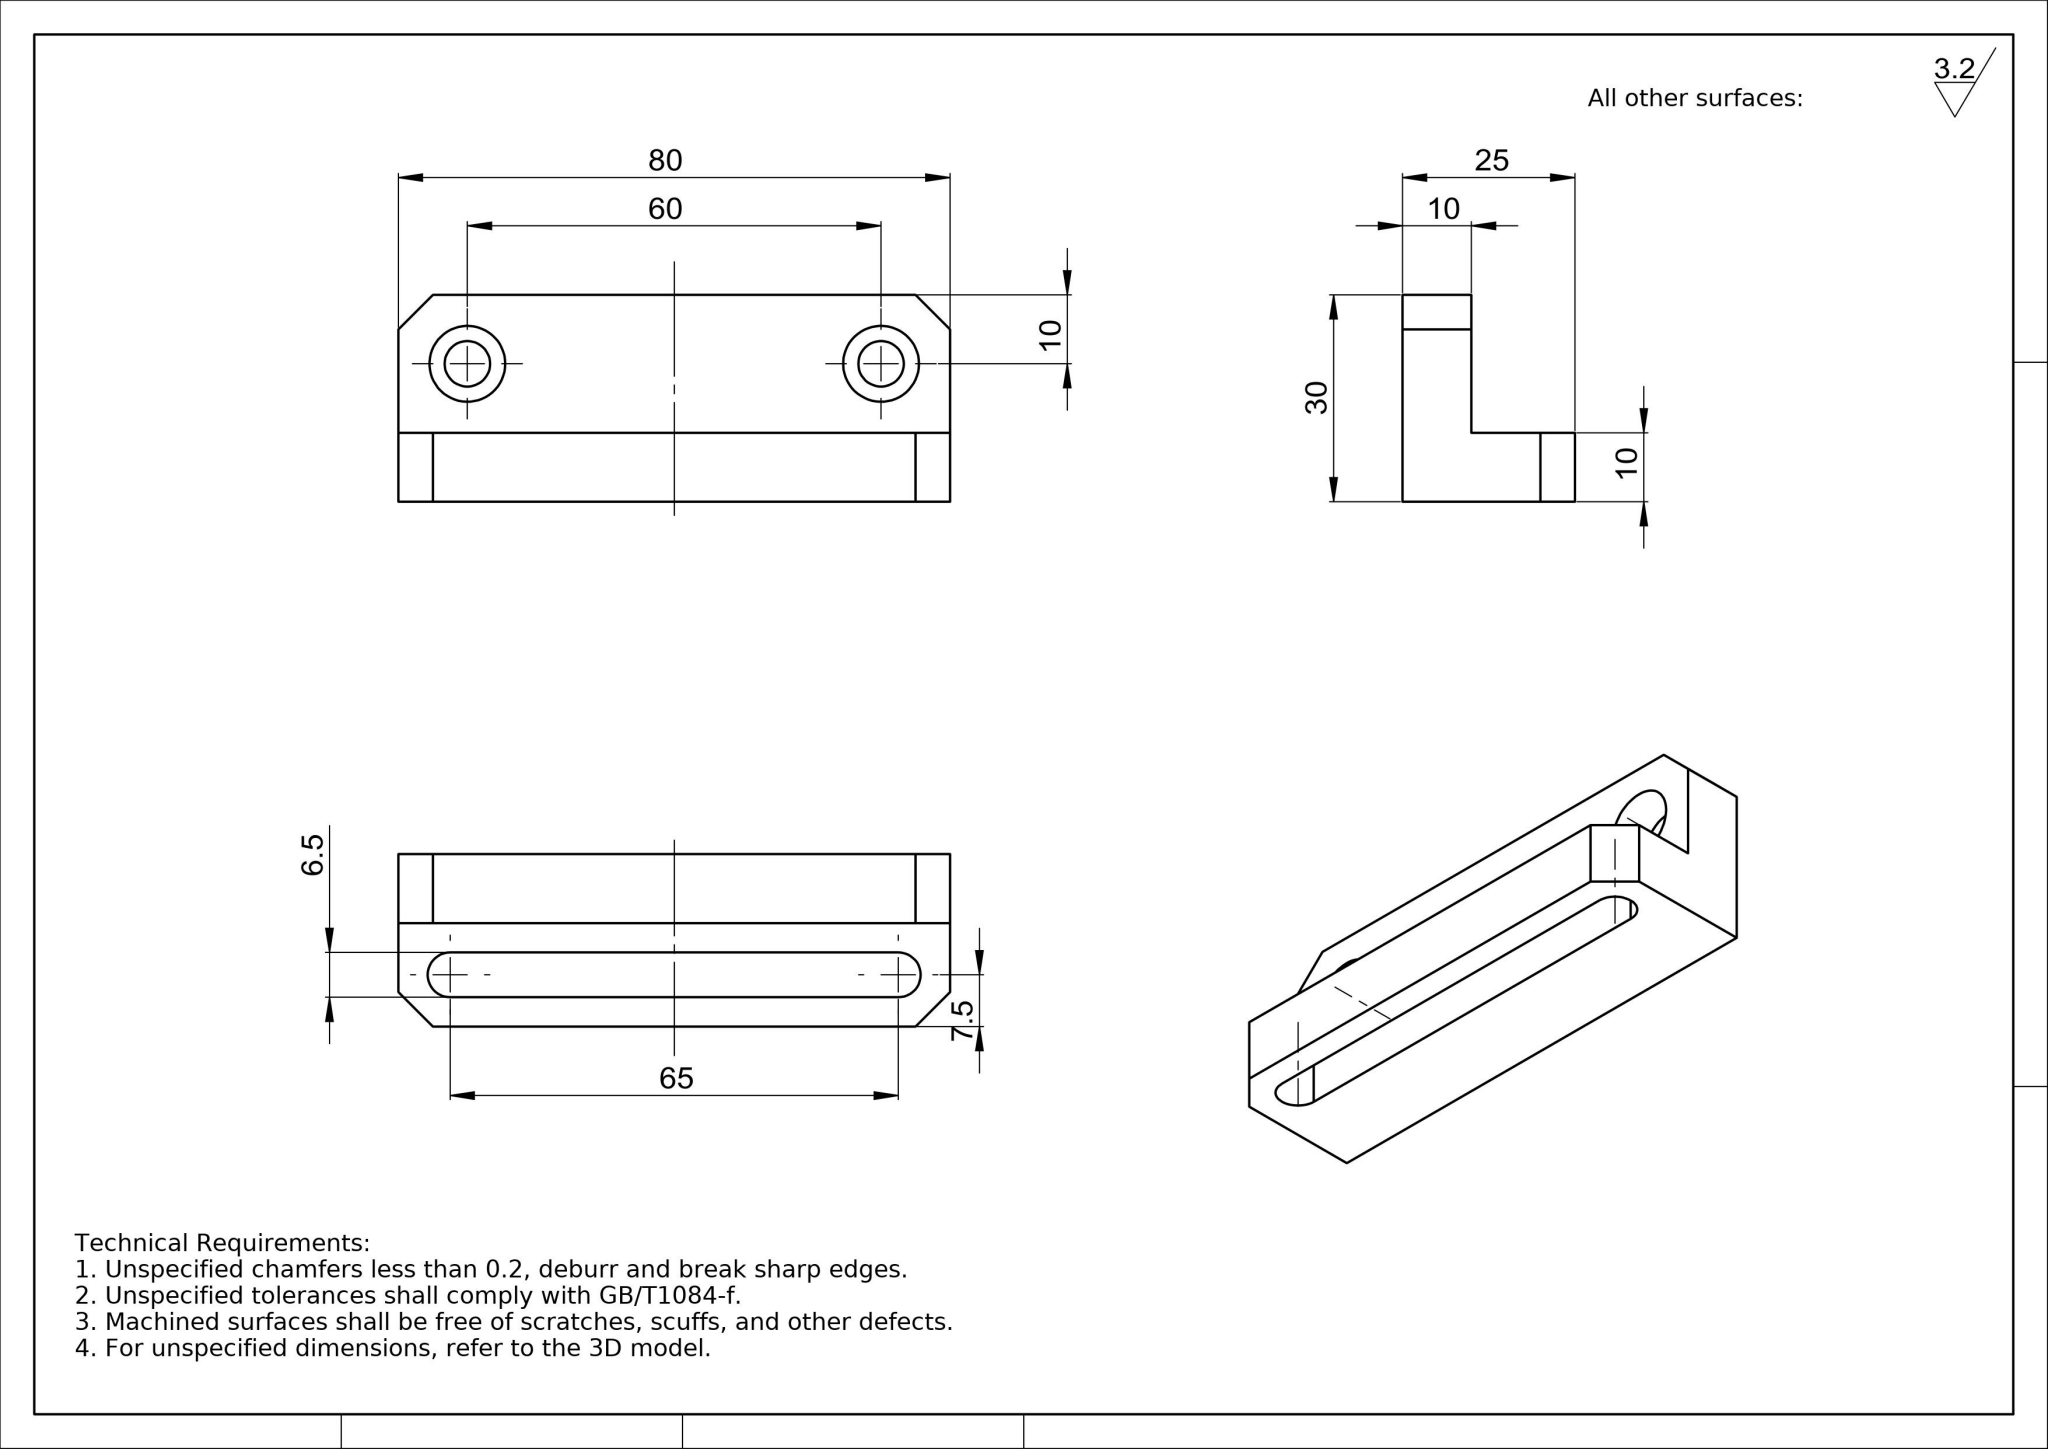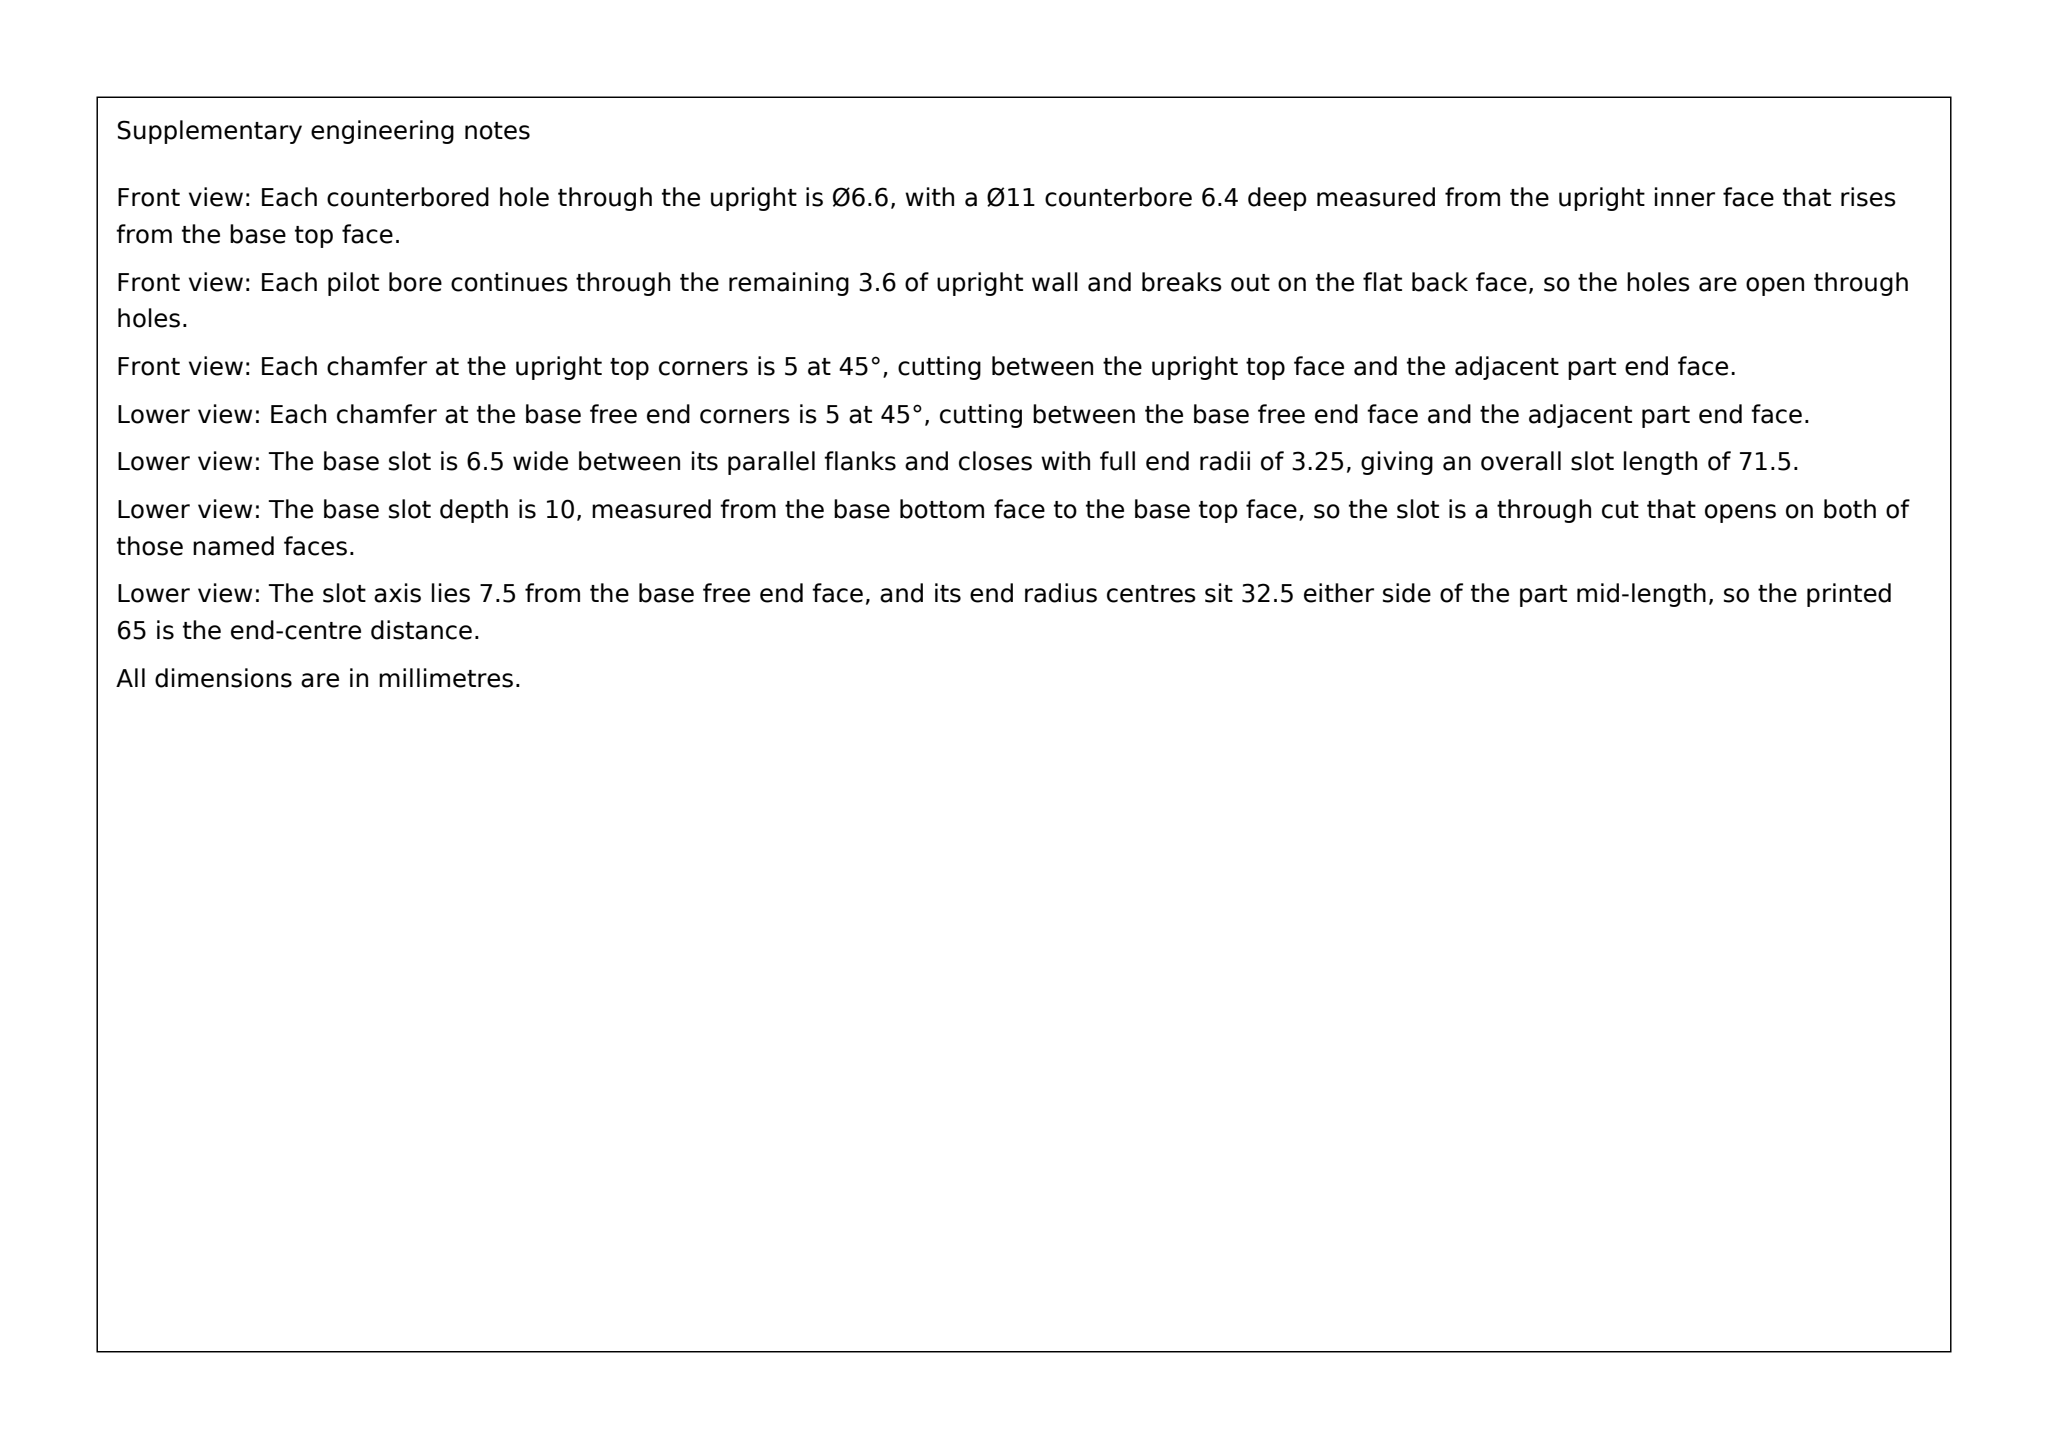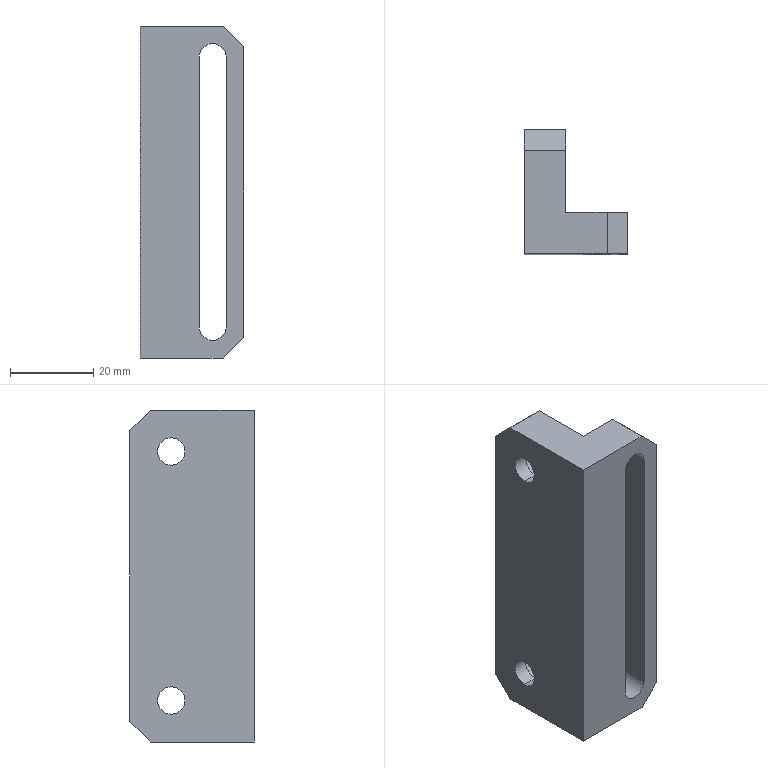Part | SolidWorks | mm | 1 solid | 26 faces | box 25 x 30 x 80 mm | volume 29480 mm3 | plane 16 | cylinder 10 | commonest cylinder face diameters 11 x4 6.6 x4 6.5 x2
Drawing notes:
SLOT 6.5 WIDE x 65 LG THRU 10 THK BASE | from the solid: Ø6.5 y-axis cyls at z=7.5 & 72.5 (65 apart), len 10 = y0 to y10 plate
2X Ø6.6 THRU, CBORE Ø11 DP 6.4 (CBORE, FLAT BTM) IN FRONT FACE | from the solid: Ø6.6 x 3.6 deep thru remaining wall + coaxial Ø11 x 6.4 flat-bottom bore, axis X, at y=20, z=10 & z=70 (10 wall)
build123d program:
from build123d import *

# Parameters (mm, degrees)
BOSS_EXTRUDE1_DEPTH                             = 40
CHAMFER1_SIZE                                   = 5
M6_HEX_SOCKET_HEAD_CAP_SCREW_CBORE1_D           = 6.6
M6_HEX_SOCKET_HEAD_CAP_SCREW_CBORE1_DEPTH       = 17.4
M6_HEX_SOCKET_HEAD_CAP_SCREW_CBORE1_CBORE_D     = 11
M6_HEX_SOCKET_HEAD_CAP_SCREW_CBORE1_CBORE_DEPTH = 6.4
M6_HEX_SOCKET_HEAD_CAP_SCREW_CBORE1_TIP         = 1.983
CUT_EXTRUDE1_DEPTH                              = 52.235


with BuildPart() as part:
    # Sketch1 → Boss-Extrude1 (new, symmetric)
    with BuildSketch(Plane.XY):
        Polygon((0, 0), (0, 30), (10, 30), (10, 10), (25, 10), (25, 0), align=None)
    extrude(amount=BOSS_EXTRUDE1_DEPTH, both=True)

    # Chamfer1
    chamfer1_edges = [part.edges().sort_by_distance(p)[0] for p in [
        (5, 30, 40),
        (5, 30, -40),
        (25, 5, -40),
        (25, 5, 40),
    ]]
    chamfer(chamfer1_edges, length=CHAMFER1_SIZE)

    # M6 Hex Socket Head Cap Screw CBORE1
    with Locations(Plane(origin=(10, 0, 0), x_dir=(0, 0, -1), z_dir=(1, 0, 0))):
        with Locations((-30, 20), (30, 20)):
            CounterBoreHole(M6_HEX_SOCKET_HEAD_CAP_SCREW_CBORE1_D / 2, M6_HEX_SOCKET_HEAD_CAP_SCREW_CBORE1_CBORE_D / 2, M6_HEX_SOCKET_HEAD_CAP_SCREW_CBORE1_CBORE_DEPTH, depth=M6_HEX_SOCKET_HEAD_CAP_SCREW_CBORE1_DEPTH)
            with Locations((0, 0, -(M6_HEX_SOCKET_HEAD_CAP_SCREW_CBORE1_DEPTH + M6_HEX_SOCKET_HEAD_CAP_SCREW_CBORE1_TIP / 2))):  # 118° drill point
                Cone(0, M6_HEX_SOCKET_HEAD_CAP_SCREW_CBORE1_D / 2, M6_HEX_SOCKET_HEAD_CAP_SCREW_CBORE1_TIP, mode=Mode.SUBTRACT)

    # Sketch4 → Cut-Extrude1 (cut, through all)
    with BuildSketch(Plane(origin=(0, 10, 0), x_dir=(1, 0, 0), z_dir=(0, 1, 0))):
        with BuildLine():
            Line((20.75, 32.5), (20.75, -32.5))
            ThreePointArc((20.75, -32.5), (17.5, -35.75), (14.25, -32.5))
            Line((14.25, -32.5), (14.25, 32.5))
            ThreePointArc((14.25, 32.5), (17.5, 35.75), (20.75, 32.5))
        make_face()
    extrude(amount=-CUT_EXTRUDE1_DEPTH, mode=Mode.SUBTRACT)


solid = part.part
STEP:
#1=CARTESIAN_POINT('',(3.6,20.,35.5));
#2=VERTEX_POINT('',#1);
#3=CARTESIAN_POINT('',(3.6,20.,24.5));
#4=VERTEX_POINT('',#3);
#5=CARTESIAN_POINT('',(3.6,20.,30.));
#6=DIRECTION('',(1.,0.,0.));
#7=DIRECTION('',(0.,0.,-1.));
#8=AXIS2_PLACEMENT_3D('',#5,#6,#7);
#9=CIRCLE('',#8,5.5);
#10=EDGE_CURVE('',#2,#4,#9,.T.);
#11=ORIENTED_EDGE('',*,*,#10,.F.);
#12=CARTESIAN_POINT('',(10.,20.,35.5));
#13=VERTEX_POINT('',#12);
#14=CARTESIAN_POINT('',(10.,20.,35.5));
#15=DIRECTION('',(1.,0.,0.));
#16=VECTOR('',#15,1000.);
#17=LINE('',#14,#16);
#18=EDGE_CURVE('',#2,#13,#17,.T.);
#19=ORIENTED_EDGE('',*,*,#18,.T.);
#20=CARTESIAN_POINT('',(10.,20.,24.5));
#21=VERTEX_POINT('',#20);
#22=CARTESIAN_POINT('',(10.,20.,30.));
#23=DIRECTION('',(1.,0.,0.));
#24=DIRECTION('',(0.,0.,-1.));
#25=AXIS2_PLACEMENT_3D('',#22,#23,#24);
#26=CIRCLE('',#25,5.5);
#27=EDGE_CURVE('',#13,#21,#26,.T.);
#28=ORIENTED_EDGE('',*,*,#27,.T.);
#29=CARTESIAN_POINT('',(10.,20.,24.5));
#30=DIRECTION('',(1.,0.,0.));
#31=VECTOR('',#30,1000.);
#32=LINE('',#29,#31);
#33=EDGE_CURVE('',#4,#21,#32,.T.);
#34=ORIENTED_EDGE('',*,*,#33,.F.);
#35=EDGE_LOOP('',(#11,#19,#28,#34));
#36=FACE_OUTER_BOUND('',#35,.T.);
#37=CARTESIAN_POINT('',(10.,20.,30.));
#38=DIRECTION('',(1.,0.,0.));
#39=DIRECTION('',(0.,0.,-1.));
#40=AXIS2_PLACEMENT_3D('',#37,#38,#39);
#41=CYLINDRICAL_SURFACE('',#40,5.5);
#42=ADVANCED_FACE('',(#36),#41,.F.);
#43=CARTESIAN_POINT('',(0.,20.,33.3));
#44=VERTEX_POINT('',#43);
#45=CARTESIAN_POINT('',(0.,20.,26.7));
#46=VERTEX_POINT('',#45);
#47=CARTESIAN_POINT('',(0.,20.,30.));
#48=DIRECTION('',(1.,0.,0.));
#49=DIRECTION('',(0.,0.,-1.));
#50=AXIS2_PLACEMENT_3D('',#47,#48,#49);
#51=CIRCLE('',#50,3.3);
#52=EDGE_CURVE('',#44,#46,#51,.T.);
#53=ORIENTED_EDGE('',*,*,#52,.F.);
#54=CARTESIAN_POINT('',(3.6,20.,33.3));
#55=VERTEX_POINT('',#54);
#56=CARTESIAN_POINT('',(10.,20.,33.3));
#57=DIRECTION('',(1.,0.,0.));
#58=VECTOR('',#57,1000.);
#59=LINE('',#56,#58);
#60=EDGE_CURVE('',#44,#55,#59,.T.);
#61=ORIENTED_EDGE('',*,*,#60,.T.);
#62=CARTESIAN_POINT('',(3.6,20.,26.7));
#63=VERTEX_POINT('',#62);
#64=CARTESIAN_POINT('',(3.6,20.,30.));
#65=DIRECTION('',(1.,0.,0.));
#66=DIRECTION('',(0.,0.,-1.));
#67=AXIS2_PLACEMENT_3D('',#64,#65,#66);
#68=CIRCLE('',#67,3.3);
#69=EDGE_CURVE('',#55,#63,#68,.T.);
#70=ORIENTED_EDGE('',*,*,#69,.T.);
#71=CARTESIAN_POINT('',(10.,20.,26.7));
#72=DIRECTION('',(1.,0.,0.));
#73=VECTOR('',#72,1000.);
#74=LINE('',#71,#73);
#75=EDGE_CURVE('',#46,#63,#74,.T.);
#76=ORIENTED_EDGE('',*,*,#75,.F.);
#77=EDGE_LOOP('',(#53,#61,#70,#76));
#78=FACE_OUTER_BOUND('',#77,.T.);
#79=CARTESIAN_POINT('',(10.,20.,30.));
#80=DIRECTION('',(1.,0.,0.));
#81=DIRECTION('',(0.,0.,-1.));
#82=AXIS2_PLACEMENT_3D('',#79,#80,#81);
#83=CYLINDRICAL_SURFACE('',#82,3.3);
#84=ADVANCED_FACE('',(#78),#83,.F.);
#85=CARTESIAN_POINT('',(3.6,20.,-24.5));
#86=VERTEX_POINT('',#85);
#87=CARTESIAN_POINT('',(3.6,20.,-35.5));
#88=VERTEX_POINT('',#87);
#89=CARTESIAN_POINT('',(3.6,20.,-30.));
#90=DIRECTION('',(1.,0.,0.));
#91=DIRECTION('',(0.,0.,-1.));
#92=AXIS2_PLACEMENT_3D('',#89,#90,#91);
#93=CIRCLE('',#92,5.5);
#94=EDGE_CURVE('',#86,#88,#93,.T.);
#95=ORIENTED_EDGE('',*,*,#94,.F.);
#96=CARTESIAN_POINT('',(10.,20.,-24.5));
#97=VERTEX_POINT('',#96);
#98=CARTESIAN_POINT('',(10.,20.,-24.5));
#99=DIRECTION('',(1.,0.,0.));
#100=VECTOR('',#99,1000.);
#101=LINE('',#98,#100);
#102=EDGE_CURVE('',#86,#97,#101,.T.);
#103=ORIENTED_EDGE('',*,*,#102,.T.);
#104=CARTESIAN_POINT('',(10.,20.,-35.5));
#105=VERTEX_POINT('',#104);
#106=CARTESIAN_POINT('',(10.,20.,-30.));
#107=DIRECTION('',(1.,0.,0.));
#108=DIRECTION('',(0.,0.,-1.));
#109=AXIS2_PLACEMENT_3D('',#106,#107,#108);
#110=CIRCLE('',#109,5.5);
#111=EDGE_CURVE('',#97,#105,#110,.T.);
#112=ORIENTED_EDGE('',*,*,#111,.T.);
#113=CARTESIAN_POINT('',(10.,20.,-35.5));
#114=DIRECTION('',(1.,0.,0.));
#115=VECTOR('',#114,1000.);
#116=LINE('',#113,#115);
#117=EDGE_CURVE('',#88,#105,#116,.T.);
#118=ORIENTED_EDGE('',*,*,#117,.F.);
#119=EDGE_LOOP('',(#95,#103,#112,#118));
#120=FACE_OUTER_BOUND('',#119,.T.);
#121=CARTESIAN_POINT('',(10.,20.,-30.));
#122=DIRECTION('',(1.,0.,0.));
#123=DIRECTION('',(0.,0.,-1.));
#124=AXIS2_PLACEMENT_3D('',#121,#122,#123);
#125=CYLINDRICAL_SURFACE('',#124,5.5);
#126=ADVANCED_FACE('',(#120),#125,.F.);
#127=CARTESIAN_POINT('',(0.,20.,-26.7));
#128=VERTEX_POINT('',#127);
#129=CARTESIAN_POINT('',(0.,20.,-33.3));
#130=VERTEX_POINT('',#129);
#131=CARTESIAN_POINT('',(0.,20.,-30.));
#132=DIRECTION('',(1.,0.,0.));
#133=DIRECTION('',(0.,0.,-1.));
#134=AXIS2_PLACEMENT_3D('',#131,#132,#133);
#135=CIRCLE('',#134,3.3);
#136=EDGE_CURVE('',#128,#130,#135,.T.);
#137=ORIENTED_EDGE('',*,*,#136,.F.);
#138=CARTESIAN_POINT('',(3.6,20.,-26.7));
#139=VERTEX_POINT('',#138);
#140=CARTESIAN_POINT('',(10.,20.,-26.7));
#141=DIRECTION('',(1.,0.,0.));
#142=VECTOR('',#141,1000.);
#143=LINE('',#140,#142);
#144=EDGE_CURVE('',#128,#139,#143,.T.);
#145=ORIENTED_EDGE('',*,*,#144,.T.);
#146=CARTESIAN_POINT('',(3.6,20.,-33.3));
#147=VERTEX_POINT('',#146);
#148=CARTESIAN_POINT('',(3.6,20.,-30.));
#149=DIRECTION('',(1.,0.,0.));
#150=DIRECTION('',(0.,0.,-1.));
#151=AXIS2_PLACEMENT_3D('',#148,#149,#150);
#152=CIRCLE('',#151,3.3);
#153=EDGE_CURVE('',#139,#147,#152,.T.);
#154=ORIENTED_EDGE('',*,*,#153,.T.);
#155=CARTESIAN_POINT('',(10.,20.,-33.3));
#156=DIRECTION('',(1.,0.,0.));
#157=VECTOR('',#156,1000.);
#158=LINE('',#155,#157);
#159=EDGE_CURVE('',#130,#147,#158,.T.);
#160=ORIENTED_EDGE('',*,*,#159,.F.);
#161=EDGE_LOOP('',(#137,#145,#154,#160));
#162=FACE_OUTER_BOUND('',#161,.T.);
#163=CARTESIAN_POINT('',(10.,20.,-30.));
#164=DIRECTION('',(1.,0.,0.));
#165=DIRECTION('',(0.,0.,-1.));
#166=AXIS2_PLACEMENT_3D('',#163,#164,#165);
#167=CYLINDRICAL_SURFACE('',#166,3.3);
#168=ADVANCED_FACE('',(#162),#167,.F.);
#169=CARTESIAN_POINT('',(20.75,-0.,32.5));
#170=VERTEX_POINT('',#169);
#171=CARTESIAN_POINT('',(20.75,-0.,-32.5));
#172=VERTEX_POINT('',#171);
#173=CARTESIAN_POINT('',(20.75,-0.,-32.5));
#174=DIRECTION('',(0.,0.,-1.));
#175=VECTOR('',#174,1000.);
#176=LINE('',#173,#175);
#177=EDGE_CURVE('',#170,#172,#176,.T.);
#178=ORIENTED_EDGE('',*,*,#177,.T.);
#179=CARTESIAN_POINT('',(14.25,-0.,-32.5));
#180=VERTEX_POINT('',#179);
#181=CARTESIAN_POINT('',(17.5,-0.,-32.5));
#182=DIRECTION('',(0.,1.,0.));
#183=DIRECTION('',(-1.,0.,0.));
#184=AXIS2_PLACEMENT_3D('',#181,#182,#183);
#185=CIRCLE('',#184,3.25);
#186=EDGE_CURVE('',#172,#180,#185,.T.);
#187=ORIENTED_EDGE('',*,*,#186,.T.);
#188=CARTESIAN_POINT('',(14.25,0.,32.5));
#189=VERTEX_POINT('',#188);
#190=CARTESIAN_POINT('',(14.25,-0.,-32.5));
#191=DIRECTION('',(0.,0.,1.));
#192=VECTOR('',#191,1000.);
#193=LINE('',#190,#192);
#194=EDGE_CURVE('',#180,#189,#193,.T.);
#195=ORIENTED_EDGE('',*,*,#194,.T.);
#196=CARTESIAN_POINT('',(17.5,-0.,32.5));
#197=DIRECTION('',(0.,1.,0.));
#198=DIRECTION('',(-1.,0.,0.));
#199=AXIS2_PLACEMENT_3D('',#196,#197,#198);
#200=CIRCLE('',#199,3.25);
#201=EDGE_CURVE('',#189,#170,#200,.T.);
#202=ORIENTED_EDGE('',*,*,#201,.T.);
#203=EDGE_LOOP('',(#178,#187,#195,#202));
#204=FACE_BOUND('',#203,.T.);
#205=CARTESIAN_POINT('',(0.,0.,-40.));
#206=VERTEX_POINT('',#205);
#207=CARTESIAN_POINT('',(20.,0.,-40.));
#208=VERTEX_POINT('',#207);
#209=CARTESIAN_POINT('',(25.,0.,-40.));
#210=DIRECTION('',(1.,0.,0.));
#211=VECTOR('',#210,1000.);
#212=LINE('',#209,#211);
#213=EDGE_CURVE('',#206,#208,#212,.T.);
#214=ORIENTED_EDGE('',*,*,#213,.T.);
#215=CARTESIAN_POINT('',(25.,0.,-35.));
#216=VERTEX_POINT('',#215);
#217=CARTESIAN_POINT('',(25.,0.,-35.));
#218=DIRECTION('',(0.7071,0.,0.7071));
#219=VECTOR('',#218,1000.);
#220=LINE('',#217,#219);
#221=EDGE_CURVE('',#208,#216,#220,.T.);
#222=ORIENTED_EDGE('',*,*,#221,.T.);
#223=CARTESIAN_POINT('',(25.,0.,35.));
#224=VERTEX_POINT('',#223);
#225=CARTESIAN_POINT('',(25.,0.,40.));
#226=DIRECTION('',(0.,0.,-1.));
#227=VECTOR('',#226,1000.);
#228=LINE('',#225,#227);
#229=EDGE_CURVE('',#224,#216,#228,.T.);
#230=ORIENTED_EDGE('',*,*,#229,.F.);
#231=CARTESIAN_POINT('',(20.,0.,40.));
#232=VERTEX_POINT('',#231);
#233=CARTESIAN_POINT('',(20.,0.,40.));
#234=DIRECTION('',(-0.7071,-0.,0.7071));
#235=VECTOR('',#234,1000.);
#236=LINE('',#233,#235);
#237=EDGE_CURVE('',#224,#232,#236,.T.);
#238=ORIENTED_EDGE('',*,*,#237,.T.);
#239=CARTESIAN_POINT('',(0.,0.,40.));
#240=VERTEX_POINT('',#239);
#241=CARTESIAN_POINT('',(25.,0.,40.));
#242=DIRECTION('',(1.,0.,0.));
#243=VECTOR('',#242,1000.);
#244=LINE('',#241,#243);
#245=EDGE_CURVE('',#240,#232,#244,.T.);
#246=ORIENTED_EDGE('',*,*,#245,.F.);
#247=CARTESIAN_POINT('',(0.,0.,40.));
#248=DIRECTION('',(0.,0.,-1.));
#249=VECTOR('',#248,1000.);
#250=LINE('',#247,#249);
#251=EDGE_CURVE('',#240,#206,#250,.T.);
#252=ORIENTED_EDGE('',*,*,#251,.T.);
#253=EDGE_LOOP('',(#214,#222,#230,#238,#246,#252));
#254=FACE_OUTER_BOUND('',#253,.T.);
#255=CARTESIAN_POINT('',(25.,0.,40.));
#256=DIRECTION('',(-0.,1.,0.));
#257=DIRECTION('',(-1.,-0.,0.));
#258=AXIS2_PLACEMENT_3D('',#255,#256,#257);
#259=PLANE('',#258);
#260=ADVANCED_FACE('',(#204,#254),#259,.F.);
#261=ORIENTED_EDGE('',*,*,#229,.T.);
#262=CARTESIAN_POINT('',(25.,10.,-35.));
#263=VERTEX_POINT('',#262);
#264=CARTESIAN_POINT('',(25.,10.,-35.));
#265=DIRECTION('',(0.,1.,0.));
#266=VECTOR('',#265,1000.);
#267=LINE('',#264,#266);
#268=EDGE_CURVE('',#216,#263,#267,.T.);
#269=ORIENTED_EDGE('',*,*,#268,.T.);
#270=CARTESIAN_POINT('',(25.,10.,35.));
#271=VERTEX_POINT('',#270);
#272=CARTESIAN_POINT('',(25.,10.,40.));
#273=DIRECTION('',(0.,0.,-1.));
#274=VECTOR('',#273,1000.);
#275=LINE('',#272,#274);
#276=EDGE_CURVE('',#271,#263,#275,.T.);
#277=ORIENTED_EDGE('',*,*,#276,.F.);
#278=CARTESIAN_POINT('',(25.,10.,35.));
#279=DIRECTION('',(0.,-1.,0.));
#280=VECTOR('',#279,1000.);
#281=LINE('',#278,#280);
#282=EDGE_CURVE('',#271,#224,#281,.T.);
#283=ORIENTED_EDGE('',*,*,#282,.T.);
#284=EDGE_LOOP('',(#261,#269,#277,#283));
#285=FACE_OUTER_BOUND('',#284,.T.);
#286=CARTESIAN_POINT('',(25.,10.,40.));
#287=DIRECTION('',(-1.,0.,0.));
#288=DIRECTION('',(0.,0.,1.));
#289=AXIS2_PLACEMENT_3D('',#286,#287,#288);
#290=PLANE('',#289);
#291=ADVANCED_FACE('',(#285),#290,.F.);
#292=CARTESIAN_POINT('',(14.25,10.,-32.5));
#293=VERTEX_POINT('',#292);
#294=CARTESIAN_POINT('',(14.25,10.,32.5));
#295=VERTEX_POINT('',#294);
#296=CARTESIAN_POINT('',(14.25,10.,-32.5));
#297=DIRECTION('',(0.,0.,1.));
#298=VECTOR('',#297,1000.);
#299=LINE('',#296,#298);
#300=EDGE_CURVE('',#293,#295,#299,.T.);
#301=ORIENTED_EDGE('',*,*,#300,.F.);
#302=CARTESIAN_POINT('',(20.75,10.,-32.5));
#303=VERTEX_POINT('',#302);
#304=CARTESIAN_POINT('',(17.5,10.,-32.5));
#305=DIRECTION('',(0.,1.,0.));
#306=DIRECTION('',(-1.,0.,0.));
#307=AXIS2_PLACEMENT_3D('',#304,#305,#306);
#308=CIRCLE('',#307,3.25);
#309=EDGE_CURVE('',#303,#293,#308,.T.);
#310=ORIENTED_EDGE('',*,*,#309,.F.);
#311=CARTESIAN_POINT('',(20.75,10.,32.5));
#312=VERTEX_POINT('',#311);
#313=CARTESIAN_POINT('',(20.75,10.,-32.5));
#314=DIRECTION('',(0.,0.,-1.));
#315=VECTOR('',#314,1000.);
#316=LINE('',#313,#315);
#317=EDGE_CURVE('',#312,#303,#316,.T.);
#318=ORIENTED_EDGE('',*,*,#317,.F.);
#319=CARTESIAN_POINT('',(17.5,10.,32.5));
#320=DIRECTION('',(0.,1.,0.));
#321=DIRECTION('',(-1.,0.,0.));
#322=AXIS2_PLACEMENT_3D('',#319,#320,#321);
#323=CIRCLE('',#322,3.25);
#324=EDGE_CURVE('',#295,#312,#323,.T.);
#325=ORIENTED_EDGE('',*,*,#324,.F.);
#326=EDGE_LOOP('',(#301,#310,#318,#325));
#327=FACE_BOUND('',#326,.T.);
#328=ORIENTED_EDGE('',*,*,#276,.T.);
#329=CARTESIAN_POINT('',(20.,10.,-40.));
#330=VERTEX_POINT('',#329);
#331=CARTESIAN_POINT('',(25.,10.,-35.));
#332=DIRECTION('',(-0.7071,0.,-0.7071));
#333=VECTOR('',#332,1000.);
#334=LINE('',#331,#333);
#335=EDGE_CURVE('',#263,#330,#334,.T.);
#336=ORIENTED_EDGE('',*,*,#335,.T.);
#337=CARTESIAN_POINT('',(10.,10.,-40.));
#338=VERTEX_POINT('',#337);
#339=CARTESIAN_POINT('',(10.,10.,-40.));
#340=DIRECTION('',(-1.,0.,0.));
#341=VECTOR('',#340,1000.);
#342=LINE('',#339,#341);
#343=EDGE_CURVE('',#330,#338,#342,.T.);
#344=ORIENTED_EDGE('',*,*,#343,.T.);
#345=CARTESIAN_POINT('',(10.,10.,40.));
#346=VERTEX_POINT('',#345);
#347=CARTESIAN_POINT('',(10.,10.,40.));
#348=DIRECTION('',(0.,0.,-1.));
#349=VECTOR('',#348,1000.);
#350=LINE('',#347,#349);
#351=EDGE_CURVE('',#346,#338,#350,.T.);
#352=ORIENTED_EDGE('',*,*,#351,.F.);
#353=CARTESIAN_POINT('',(20.,10.,40.));
#354=VERTEX_POINT('',#353);
#355=CARTESIAN_POINT('',(10.,10.,40.));
#356=DIRECTION('',(-1.,0.,0.));
#357=VECTOR('',#356,1000.);
#358=LINE('',#355,#357);
#359=EDGE_CURVE('',#354,#346,#358,.T.);
#360=ORIENTED_EDGE('',*,*,#359,.F.);
#361=CARTESIAN_POINT('',(20.,10.,40.));
#362=DIRECTION('',(0.7071,-0.,-0.7071));
#363=VECTOR('',#362,1000.);
#364=LINE('',#361,#363);
#365=EDGE_CURVE('',#354,#271,#364,.T.);
#366=ORIENTED_EDGE('',*,*,#365,.T.);
#367=EDGE_LOOP('',(#328,#336,#344,#352,#360,#366));
#368=FACE_OUTER_BOUND('',#367,.T.);
#369=CARTESIAN_POINT('',(10.,10.,40.));
#370=DIRECTION('',(-0.,-1.,0.));
#371=DIRECTION('',(1.,-0.,0.));
#372=AXIS2_PLACEMENT_3D('',#369,#370,#371);
#373=PLANE('',#372);
#374=ADVANCED_FACE('',(#327,#368),#373,.F.);
#375=CARTESIAN_POINT('',(10.,20.,30.));
#376=DIRECTION('',(1.,0.,0.));
#377=DIRECTION('',(0.,0.,-1.));
#378=AXIS2_PLACEMENT_3D('',#375,#376,#377);
#379=CIRCLE('',#378,5.5);
#380=EDGE_CURVE('',#21,#13,#379,.T.);
#381=ORIENTED_EDGE('',*,*,#380,.F.);
#382=ORIENTED_EDGE('',*,*,#27,.F.);
#383=EDGE_LOOP('',(#381,#382));
#384=FACE_BOUND('',#383,.T.);
#385=CARTESIAN_POINT('',(10.,20.,-30.));
#386=DIRECTION('',(1.,0.,0.));
#387=DIRECTION('',(0.,0.,-1.));
#388=AXIS2_PLACEMENT_3D('',#385,#386,#387);
#389=CIRCLE('',#388,5.5);
#390=EDGE_CURVE('',#105,#97,#389,.T.);
#391=ORIENTED_EDGE('',*,*,#390,.F.);
#392=ORIENTED_EDGE('',*,*,#111,.F.);
#393=EDGE_LOOP('',(#391,#392));
#394=FACE_BOUND('',#393,.T.);
#395=CARTESIAN_POINT('',(10.,25.,-40.));
#396=VERTEX_POINT('',#395);
#397=CARTESIAN_POINT('',(10.,30.,-40.));
#398=DIRECTION('',(0.,1.,0.));
#399=VECTOR('',#398,1000.);
#400=LINE('',#397,#399);
#401=EDGE_CURVE('',#338,#396,#400,.T.);
#402=ORIENTED_EDGE('',*,*,#401,.T.);
#403=CARTESIAN_POINT('',(10.,30.,-35.));
#404=VERTEX_POINT('',#403);
#405=CARTESIAN_POINT('',(10.,30.,-35.));
#406=DIRECTION('',(0.,0.7071,0.7071));
#407=VECTOR('',#406,1000.);
#408=LINE('',#405,#407);
#409=EDGE_CURVE('',#396,#404,#408,.T.);
#410=ORIENTED_EDGE('',*,*,#409,.T.);
#411=CARTESIAN_POINT('',(10.,30.,35.));
#412=VERTEX_POINT('',#411);
#413=CARTESIAN_POINT('',(10.,30.,40.));
#414=DIRECTION('',(0.,0.,-1.));
#415=VECTOR('',#414,1000.);
#416=LINE('',#413,#415);
#417=EDGE_CURVE('',#412,#404,#416,.T.);
#418=ORIENTED_EDGE('',*,*,#417,.F.);
#419=CARTESIAN_POINT('',(10.,25.,40.));
#420=VERTEX_POINT('',#419);
#421=CARTESIAN_POINT('',(10.,25.,40.));
#422=DIRECTION('',(0.,-0.7071,0.7071));
#423=VECTOR('',#422,1000.);
#424=LINE('',#421,#423);
#425=EDGE_CURVE('',#412,#420,#424,.T.);
#426=ORIENTED_EDGE('',*,*,#425,.T.);
#427=CARTESIAN_POINT('',(10.,30.,40.));
#428=DIRECTION('',(0.,1.,0.));
#429=VECTOR('',#428,1000.);
#430=LINE('',#427,#429);
#431=EDGE_CURVE('',#346,#420,#430,.T.);
#432=ORIENTED_EDGE('',*,*,#431,.F.);
#433=ORIENTED_EDGE('',*,*,#351,.T.);
#434=EDGE_LOOP('',(#402,#410,#418,#426,#432,#433));
#435=FACE_OUTER_BOUND('',#434,.T.);
#436=CARTESIAN_POINT('',(10.,30.,40.));
#437=DIRECTION('',(-1.,0.,0.));
#438=DIRECTION('',(0.,0.,1.));
#439=AXIS2_PLACEMENT_3D('',#436,#437,#438);
#440=PLANE('',#439);
#441=ADVANCED_FACE('',(#384,#394,#435),#440,.F.);
#442=ORIENTED_EDGE('',*,*,#417,.T.);
#443=CARTESIAN_POINT('',(0.,30.,-35.));
#444=VERTEX_POINT('',#443);
#445=CARTESIAN_POINT('',(0.,30.,-35.));
#446=DIRECTION('',(-1.,0.,0.));
#447=VECTOR('',#446,1000.);
#448=LINE('',#445,#447);
#449=EDGE_CURVE('',#404,#444,#448,.T.);
#450=ORIENTED_EDGE('',*,*,#449,.T.);
#451=CARTESIAN_POINT('',(0.,30.,35.));
#452=VERTEX_POINT('',#451);
#453=CARTESIAN_POINT('',(0.,30.,40.));
#454=DIRECTION('',(0.,0.,-1.));
#455=VECTOR('',#454,1000.);
#456=LINE('',#453,#455);
#457=EDGE_CURVE('',#452,#444,#456,.T.);
#458=ORIENTED_EDGE('',*,*,#457,.F.);
#459=CARTESIAN_POINT('',(0.,30.,35.));
#460=DIRECTION('',(1.,0.,0.));
#461=VECTOR('',#460,1000.);
#462=LINE('',#459,#461);
#463=EDGE_CURVE('',#452,#412,#462,.T.);
#464=ORIENTED_EDGE('',*,*,#463,.T.);
#465=EDGE_LOOP('',(#442,#450,#458,#464));
#466=FACE_OUTER_BOUND('',#465,.T.);
#467=CARTESIAN_POINT('',(0.,30.,40.));
#468=DIRECTION('',(0.,-1.,0.));
#469=DIRECTION('',(0.,0.,-1.));
#470=AXIS2_PLACEMENT_3D('',#467,#468,#469);
#471=PLANE('',#470);
#472=ADVANCED_FACE('',(#466),#471,.F.);
#473=CARTESIAN_POINT('',(0.,20.,30.));
#474=DIRECTION('',(1.,0.,0.));
#475=DIRECTION('',(0.,0.,-1.));
#476=AXIS2_PLACEMENT_3D('',#473,#474,#475);
#477=CIRCLE('',#476,3.3);
#478=EDGE_CURVE('',#46,#44,#477,.T.);
#479=ORIENTED_EDGE('',*,*,#478,.T.);
#480=ORIENTED_EDGE('',*,*,#52,.T.);
#481=EDGE_LOOP('',(#479,#480));
#482=FACE_BOUND('',#481,.T.);
#483=CARTESIAN_POINT('',(0.,20.,-30.));
#484=DIRECTION('',(1.,0.,0.));
#485=DIRECTION('',(0.,0.,-1.));
#486=AXIS2_PLACEMENT_3D('',#483,#484,#485);
#487=CIRCLE('',#486,3.3);
#488=EDGE_CURVE('',#130,#128,#487,.T.);
#489=ORIENTED_EDGE('',*,*,#488,.T.);
#490=ORIENTED_EDGE('',*,*,#136,.T.);
#491=EDGE_LOOP('',(#489,#490));
#492=FACE_BOUND('',#491,.T.);
#493=ORIENTED_EDGE('',*,*,#457,.T.);
#494=CARTESIAN_POINT('',(0.,25.,-40.));
#495=VERTEX_POINT('',#494);
#496=CARTESIAN_POINT('',(0.,30.,-35.));
#497=DIRECTION('',(0.,-0.7071,-0.7071));
#498=VECTOR('',#497,1000.);
#499=LINE('',#496,#498);
#500=EDGE_CURVE('',#444,#495,#499,.T.);
#501=ORIENTED_EDGE('',*,*,#500,.T.);
#502=CARTESIAN_POINT('',(0.,0.,-40.));
#503=DIRECTION('',(0.,-1.,0.));
#504=VECTOR('',#503,1000.);
#505=LINE('',#502,#504);
#506=EDGE_CURVE('',#495,#206,#505,.T.);
#507=ORIENTED_EDGE('',*,*,#506,.T.);
#508=ORIENTED_EDGE('',*,*,#251,.F.);
#509=CARTESIAN_POINT('',(0.,25.,40.));
#510=VERTEX_POINT('',#509);
#511=CARTESIAN_POINT('',(0.,0.,40.));
#512=DIRECTION('',(0.,-1.,0.));
#513=VECTOR('',#512,1000.);
#514=LINE('',#511,#513);
#515=EDGE_CURVE('',#510,#240,#514,.T.);
#516=ORIENTED_EDGE('',*,*,#515,.F.);
#517=CARTESIAN_POINT('',(0.,25.,40.));
#518=DIRECTION('',(0.,0.7071,-0.7071));
#519=VECTOR('',#518,1000.);
#520=LINE('',#517,#519);
#521=EDGE_CURVE('',#510,#452,#520,.T.);
#522=ORIENTED_EDGE('',*,*,#521,.T.);
#523=EDGE_LOOP('',(#493,#501,#507,#508,#516,#522));
#524=FACE_OUTER_BOUND('',#523,.T.);
#525=CARTESIAN_POINT('',(0.,0.,40.));
#526=DIRECTION('',(1.,0.,0.));
#527=DIRECTION('',(0.,0.,-1.));
#528=AXIS2_PLACEMENT_3D('',#525,#526,#527);
#529=PLANE('',#528);
#530=ADVANCED_FACE('',(#482,#492,#524),#529,.F.);
#531=ORIENTED_EDGE('',*,*,#245,.T.);
#532=CARTESIAN_POINT('',(20.,0.,40.));
#533=DIRECTION('',(0.,1.,0.));
#534=VECTOR('',#533,1000.);
#535=LINE('',#532,#534);
#536=EDGE_CURVE('',#232,#354,#535,.T.);
#537=ORIENTED_EDGE('',*,*,#536,.T.);
#538=ORIENTED_EDGE('',*,*,#359,.T.);
#539=ORIENTED_EDGE('',*,*,#431,.T.);
#540=CARTESIAN_POINT('',(0.,25.,40.));
#541=DIRECTION('',(-1.,0.,0.));
#542=VECTOR('',#541,1000.);
#543=LINE('',#540,#542);
#544=EDGE_CURVE('',#420,#510,#543,.T.);
#545=ORIENTED_EDGE('',*,*,#544,.T.);
#546=ORIENTED_EDGE('',*,*,#515,.T.);
#547=EDGE_LOOP('',(#531,#537,#538,#539,#545,#546));
#548=FACE_OUTER_BOUND('',#547,.T.);
#549=CARTESIAN_POINT('',(0.,0.,40.));
#550=DIRECTION('',(0.,0.,-1.));
#551=DIRECTION('',(-1.,0.,0.));
#552=AXIS2_PLACEMENT_3D('',#549,#550,#551);
#553=PLANE('',#552);
#554=ADVANCED_FACE('',(#548),#553,.F.);
#555=ORIENTED_EDGE('',*,*,#343,.F.);
#556=CARTESIAN_POINT('',(20.,0.,-40.));
#557=DIRECTION('',(0.,-1.,0.));
#558=VECTOR('',#557,1000.);
#559=LINE('',#556,#558);
#560=EDGE_CURVE('',#330,#208,#559,.T.);
#561=ORIENTED_EDGE('',*,*,#560,.T.);
#562=ORIENTED_EDGE('',*,*,#213,.F.);
#563=ORIENTED_EDGE('',*,*,#506,.F.);
#564=CARTESIAN_POINT('',(10.,25.,-40.));
#565=DIRECTION('',(1.,0.,0.));
#566=VECTOR('',#565,1000.);
#567=LINE('',#564,#566);
#568=EDGE_CURVE('',#495,#396,#567,.T.);
#569=ORIENTED_EDGE('',*,*,#568,.T.);
#570=ORIENTED_EDGE('',*,*,#401,.F.);
#571=EDGE_LOOP('',(#555,#561,#562,#563,#569,#570));
#572=FACE_OUTER_BOUND('',#571,.T.);
#573=CARTESIAN_POINT('',(0.,0.,-40.));
#574=DIRECTION('',(0.,0.,-1.));
#575=DIRECTION('',(-1.,0.,0.));
#576=AXIS2_PLACEMENT_3D('',#573,#574,#575);
#577=PLANE('',#576);
#578=ADVANCED_FACE('',(#572),#577,.T.);
#579=ORIENTED_EDGE('',*,*,#221,.F.);
#580=ORIENTED_EDGE('',*,*,#560,.F.);
#581=ORIENTED_EDGE('',*,*,#335,.F.);
#582=ORIENTED_EDGE('',*,*,#268,.F.);
#583=EDGE_LOOP('',(#579,#580,#581,#582));
#584=FACE_OUTER_BOUND('',#583,.T.);
#585=CARTESIAN_POINT('',(25.,10.,-35.));
#586=DIRECTION('',(0.7071,0.,-0.7071));
#587=DIRECTION('',(0.,-1.,0.));
#588=AXIS2_PLACEMENT_3D('',#585,#586,#587);
#589=PLANE('',#588);
#590=ADVANCED_FACE('',(#584),#589,.T.);
#591=ORIENTED_EDGE('',*,*,#237,.F.);
#592=ORIENTED_EDGE('',*,*,#282,.F.);
#593=ORIENTED_EDGE('',*,*,#365,.F.);
#594=ORIENTED_EDGE('',*,*,#536,.F.);
#595=EDGE_LOOP('',(#591,#592,#593,#594));
#596=FACE_OUTER_BOUND('',#595,.T.);
#597=CARTESIAN_POINT('',(20.,0.,40.));
#598=DIRECTION('',(-0.7071,0.,-0.7071));
#599=DIRECTION('',(0.,1.,0.));
#600=AXIS2_PLACEMENT_3D('',#597,#598,#599);
#601=PLANE('',#600);
#602=ADVANCED_FACE('',(#596),#601,.F.);
#603=ORIENTED_EDGE('',*,*,#409,.F.);
#604=ORIENTED_EDGE('',*,*,#568,.F.);
#605=ORIENTED_EDGE('',*,*,#500,.F.);
#606=ORIENTED_EDGE('',*,*,#449,.F.);
#607=EDGE_LOOP('',(#603,#604,#605,#606));
#608=FACE_OUTER_BOUND('',#607,.T.);
#609=CARTESIAN_POINT('',(0.,30.,-35.));
#610=DIRECTION('',(0.,0.7071,-0.7071));
#611=DIRECTION('',(1.,0.,0.));
#612=AXIS2_PLACEMENT_3D('',#609,#610,#611);
#613=PLANE('',#612);
#614=ADVANCED_FACE('',(#608),#613,.T.);
#615=ORIENTED_EDGE('',*,*,#425,.F.);
#616=ORIENTED_EDGE('',*,*,#463,.F.);
#617=ORIENTED_EDGE('',*,*,#521,.F.);
#618=ORIENTED_EDGE('',*,*,#544,.F.);
#619=EDGE_LOOP('',(#615,#616,#617,#618));
#620=FACE_OUTER_BOUND('',#619,.T.);
#621=CARTESIAN_POINT('',(0.,25.,40.));
#622=DIRECTION('',(0.,-0.7071,-0.7071));
#623=DIRECTION('',(-1.,0.,0.));
#624=AXIS2_PLACEMENT_3D('',#621,#622,#623);
#625=PLANE('',#624);
#626=ADVANCED_FACE('',(#620),#625,.F.);
#627=ORIENTED_EDGE('',*,*,#144,.F.);
#628=ORIENTED_EDGE('',*,*,#488,.F.);
#629=ORIENTED_EDGE('',*,*,#159,.T.);
#630=CARTESIAN_POINT('',(3.6,20.,-30.));
#631=DIRECTION('',(1.,0.,0.));
#632=DIRECTION('',(0.,0.,-1.));
#633=AXIS2_PLACEMENT_3D('',#630,#631,#632);
#634=CIRCLE('',#633,3.3);
#635=EDGE_CURVE('',#147,#139,#634,.T.);
#636=ORIENTED_EDGE('',*,*,#635,.T.);
#637=EDGE_LOOP('',(#627,#628,#629,#636));
#638=FACE_OUTER_BOUND('',#637,.T.);
#639=CARTESIAN_POINT('',(10.,20.,-30.));
#640=DIRECTION('',(1.,0.,0.));
#641=DIRECTION('',(0.,0.,-1.));
#642=AXIS2_PLACEMENT_3D('',#639,#640,#641);
#643=CYLINDRICAL_SURFACE('',#642,3.3);
#644=ADVANCED_FACE('',(#638),#643,.F.);
#645=ORIENTED_EDGE('',*,*,#635,.F.);
#646=ORIENTED_EDGE('',*,*,#153,.F.);
#647=EDGE_LOOP('',(#645,#646));
#648=FACE_BOUND('',#647,.T.);
#649=CARTESIAN_POINT('',(3.6,20.,-30.));
#650=DIRECTION('',(1.,0.,0.));
#651=DIRECTION('',(0.,0.,-1.));
#652=AXIS2_PLACEMENT_3D('',#649,#650,#651);
#653=CIRCLE('',#652,5.5);
#654=EDGE_CURVE('',#88,#86,#653,.T.);
#655=ORIENTED_EDGE('',*,*,#654,.T.);
#656=ORIENTED_EDGE('',*,*,#94,.T.);
#657=EDGE_LOOP('',(#655,#656));
#658=FACE_OUTER_BOUND('',#657,.T.);
#659=CARTESIAN_POINT('',(3.6,23.3,-30.));
#660=DIRECTION('',(-1.,0.,0.));
#661=DIRECTION('',(0.,0.,1.));
#662=AXIS2_PLACEMENT_3D('',#659,#660,#661);
#663=PLANE('',#662);
#664=ADVANCED_FACE('',(#648,#658),#663,.F.);
#665=ORIENTED_EDGE('',*,*,#102,.F.);
#666=ORIENTED_EDGE('',*,*,#654,.F.);
#667=ORIENTED_EDGE('',*,*,#117,.T.);
#668=ORIENTED_EDGE('',*,*,#390,.T.);
#669=EDGE_LOOP('',(#665,#666,#667,#668));
#670=FACE_OUTER_BOUND('',#669,.T.);
#671=CARTESIAN_POINT('',(10.,20.,-30.));
#672=DIRECTION('',(1.,0.,0.));
#673=DIRECTION('',(0.,0.,-1.));
#674=AXIS2_PLACEMENT_3D('',#671,#672,#673);
#675=CYLINDRICAL_SURFACE('',#674,5.5);
#676=ADVANCED_FACE('',(#670),#675,.F.);
#677=ORIENTED_EDGE('',*,*,#60,.F.);
#678=ORIENTED_EDGE('',*,*,#478,.F.);
#679=ORIENTED_EDGE('',*,*,#75,.T.);
#680=CARTESIAN_POINT('',(3.6,20.,30.));
#681=DIRECTION('',(1.,0.,0.));
#682=DIRECTION('',(0.,0.,-1.));
#683=AXIS2_PLACEMENT_3D('',#680,#681,#682);
#684=CIRCLE('',#683,3.3);
#685=EDGE_CURVE('',#63,#55,#684,.T.);
#686=ORIENTED_EDGE('',*,*,#685,.T.);
#687=EDGE_LOOP('',(#677,#678,#679,#686));
#688=FACE_OUTER_BOUND('',#687,.T.);
#689=CARTESIAN_POINT('',(10.,20.,30.));
#690=DIRECTION('',(1.,0.,0.));
#691=DIRECTION('',(0.,0.,-1.));
#692=AXIS2_PLACEMENT_3D('',#689,#690,#691);
#693=CYLINDRICAL_SURFACE('',#692,3.3);
#694=ADVANCED_FACE('',(#688),#693,.F.);
#695=ORIENTED_EDGE('',*,*,#685,.F.);
#696=ORIENTED_EDGE('',*,*,#69,.F.);
#697=EDGE_LOOP('',(#695,#696));
#698=FACE_BOUND('',#697,.T.);
#699=CARTESIAN_POINT('',(3.6,20.,30.));
#700=DIRECTION('',(1.,0.,0.));
#701=DIRECTION('',(0.,0.,-1.));
#702=AXIS2_PLACEMENT_3D('',#699,#700,#701);
#703=CIRCLE('',#702,5.5);
#704=EDGE_CURVE('',#4,#2,#703,.T.);
#705=ORIENTED_EDGE('',*,*,#704,.T.);
#706=ORIENTED_EDGE('',*,*,#10,.T.);
#707=EDGE_LOOP('',(#705,#706));
#708=FACE_OUTER_BOUND('',#707,.T.);
#709=CARTESIAN_POINT('',(3.6,23.3,30.));
#710=DIRECTION('',(-1.,0.,0.));
#711=DIRECTION('',(0.,0.,1.));
#712=AXIS2_PLACEMENT_3D('',#709,#710,#711);
#713=PLANE('',#712);
#714=ADVANCED_FACE('',(#698,#708),#713,.F.);
#715=ORIENTED_EDGE('',*,*,#18,.F.);
#716=ORIENTED_EDGE('',*,*,#704,.F.);
#717=ORIENTED_EDGE('',*,*,#33,.T.);
#718=ORIENTED_EDGE('',*,*,#380,.T.);
#719=EDGE_LOOP('',(#715,#716,#717,#718));
#720=FACE_OUTER_BOUND('',#719,.T.);
#721=CARTESIAN_POINT('',(10.,20.,30.));
#722=DIRECTION('',(1.,0.,0.));
#723=DIRECTION('',(0.,0.,-1.));
#724=AXIS2_PLACEMENT_3D('',#721,#722,#723);
#725=CYLINDRICAL_SURFACE('',#724,5.5);
#726=ADVANCED_FACE('',(#720),#725,.F.);
#727=ORIENTED_EDGE('',*,*,#309,.T.);
#728=CARTESIAN_POINT('',(14.25,-0.,-32.5));
#729=DIRECTION('',(0.,1.,0.));
#730=VECTOR('',#729,1000.);
#731=LINE('',#728,#730);
#732=EDGE_CURVE('',#180,#293,#731,.T.);
#733=ORIENTED_EDGE('',*,*,#732,.F.);
#734=ORIENTED_EDGE('',*,*,#186,.F.);
#735=CARTESIAN_POINT('',(20.75,-0.,-32.5));
#736=DIRECTION('',(0.,1.,0.));
#737=VECTOR('',#736,1000.);
#738=LINE('',#735,#737);
#739=EDGE_CURVE('',#172,#303,#738,.T.);
#740=ORIENTED_EDGE('',*,*,#739,.T.);
#741=EDGE_LOOP('',(#727,#733,#734,#740));
#742=FACE_OUTER_BOUND('',#741,.T.);
#743=CARTESIAN_POINT('',(17.5,-0.,-32.5));
#744=DIRECTION('',(0.,1.,0.));
#745=DIRECTION('',(-1.,0.,0.));
#746=AXIS2_PLACEMENT_3D('',#743,#744,#745);
#747=CYLINDRICAL_SURFACE('',#746,3.25);
#748=ADVANCED_FACE('',(#742),#747,.F.);
#749=ORIENTED_EDGE('',*,*,#317,.T.);
#750=ORIENTED_EDGE('',*,*,#739,.F.);
#751=ORIENTED_EDGE('',*,*,#177,.F.);
#752=CARTESIAN_POINT('',(20.75,-0.,32.5));
#753=DIRECTION('',(0.,1.,0.));
#754=VECTOR('',#753,1000.);
#755=LINE('',#752,#754);
#756=EDGE_CURVE('',#170,#312,#755,.T.);
#757=ORIENTED_EDGE('',*,*,#756,.T.);
#758=EDGE_LOOP('',(#749,#750,#751,#757));
#759=FACE_OUTER_BOUND('',#758,.T.);
#760=CARTESIAN_POINT('',(20.75,-0.,-32.5));
#761=DIRECTION('',(1.,-0.,0.));
#762=DIRECTION('',(0.,1.,0.));
#763=AXIS2_PLACEMENT_3D('',#760,#761,#762);
#764=PLANE('',#763);
#765=ADVANCED_FACE('',(#759),#764,.F.);
#766=ORIENTED_EDGE('',*,*,#324,.T.);
#767=ORIENTED_EDGE('',*,*,#756,.F.);
#768=ORIENTED_EDGE('',*,*,#201,.F.);
#769=CARTESIAN_POINT('',(14.25,-0.,32.5));
#770=DIRECTION('',(0.,1.,0.));
#771=VECTOR('',#770,1000.);
#772=LINE('',#769,#771);
#773=EDGE_CURVE('',#189,#295,#772,.T.);
#774=ORIENTED_EDGE('',*,*,#773,.T.);
#775=EDGE_LOOP('',(#766,#767,#768,#774));
#776=FACE_OUTER_BOUND('',#775,.T.);
#777=CARTESIAN_POINT('',(17.5,-0.,32.5));
#778=DIRECTION('',(0.,1.,0.));
#779=DIRECTION('',(-1.,0.,0.));
#780=AXIS2_PLACEMENT_3D('',#777,#778,#779);
#781=CYLINDRICAL_SURFACE('',#780,3.25);
#782=ADVANCED_FACE('',(#776),#781,.F.);
#783=ORIENTED_EDGE('',*,*,#300,.T.);
#784=ORIENTED_EDGE('',*,*,#773,.F.);
#785=ORIENTED_EDGE('',*,*,#194,.F.);
#786=ORIENTED_EDGE('',*,*,#732,.T.);
#787=EDGE_LOOP('',(#783,#784,#785,#786));
#788=FACE_OUTER_BOUND('',#787,.T.);
#789=CARTESIAN_POINT('',(14.25,-0.,-32.5));
#790=DIRECTION('',(-1.,0.,0.));
#791=DIRECTION('',(-0.,-1.,0.));
#792=AXIS2_PLACEMENT_3D('',#789,#790,#791);
#793=PLANE('',#792);
#794=ADVANCED_FACE('',(#788),#793,.F.);
#795=CLOSED_SHELL('',(#42,#84,#126,#168,#260,#291,#374,#441,#472,#530,#554,#578,#590,#602,#614,#626,#644,#664,#676,#694,#714,#726,#748,#765,#782,#794));
#796=MANIFOLD_SOLID_BREP('',#795);
#797=CARTESIAN_POINT('',(0.,0.,0.));
#798=DIRECTION('',(0.,0.,1.));
#799=DIRECTION('',(1.,0.,0.));
#800=AXIS2_PLACEMENT_3D('',#797,#798,#799);
#801=(LENGTH_UNIT()NAMED_UNIT(*)SI_UNIT(.MILLI.,.METRE.));
#802=UNCERTAINTY_MEASURE_WITH_UNIT(LENGTH_MEASURE(0.00001),#801,'','');
#803=(NAMED_UNIT(*)PLANE_ANGLE_UNIT()SI_UNIT($,.RADIAN.));
#804=(NAMED_UNIT(*)SI_UNIT($,.STERADIAN.)SOLID_ANGLE_UNIT());
#805=(GEOMETRIC_REPRESENTATION_CONTEXT(3)GLOBAL_UNCERTAINTY_ASSIGNED_CONTEXT((#802))GLOBAL_UNIT_ASSIGNED_CONTEXT((#801,#803,#804))REPRESENTATION_CONTEXT('',''));
#806=ADVANCED_BREP_SHAPE_REPRESENTATION('',(#796,#800),#805);